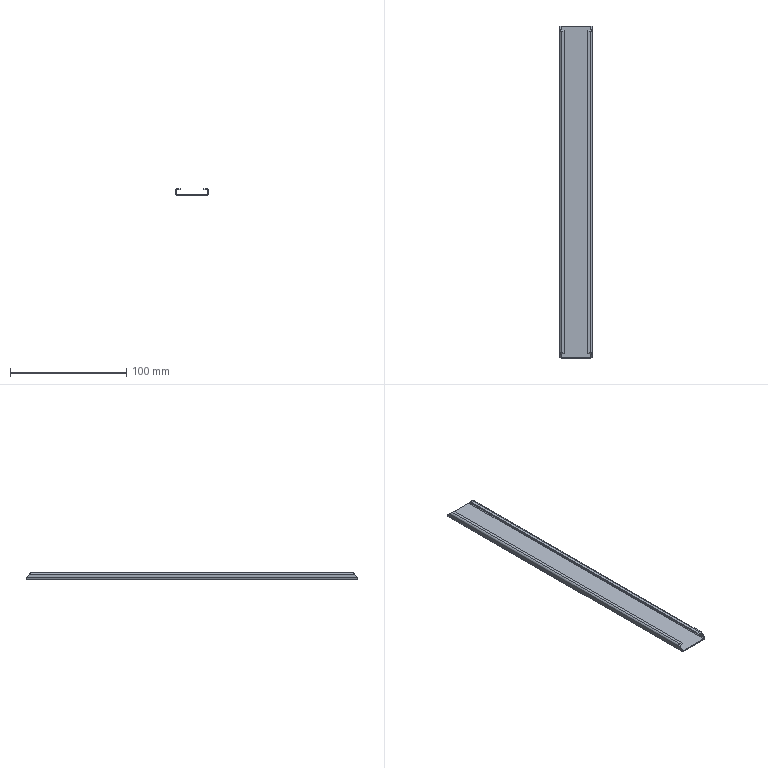Component | SolidWorks | PC-CAJ-P09-1_PM-CAJ-P55-2 | 1 solid | 30 faces | box 28 x 285 x 6 mm | volume 11970 mm3 | plane 22 | cylinder 8 | commonest cylinder face diameters 3 x4 1 x4 | material Plain Carbon Steel
STEP:
#1=COLOUR_RGB('',0.7922,0.8196,0.9333);
#2=FILL_AREA_STYLE_COLOUR('',#1);
#3=FILL_AREA_STYLE('',(#2));
#4=SURFACE_STYLE_FILL_AREA(#3);
#5=SURFACE_SIDE_STYLE('',(#4));
#6=SURFACE_STYLE_USAGE(.BOTH.,#5);
#7=PRESENTATION_STYLE_ASSIGNMENT((#6));
#8=CARTESIAN_POINT('',(6.496,0.5209,3.209));
#9=VERTEX_POINT('',#8);
#10=CARTESIAN_POINT('',(6.496,0.4815,3.169));
#11=VERTEX_POINT('',#10);
#12=CARTESIAN_POINT('',(6.496,0.5209,3.209));
#13=DIRECTION('',(0.,-0.7071,-0.7071));
#14=VECTOR('',#13,39.37);
#15=LINE('',#12,#14);
#16=EDGE_CURVE('',#9,#11,#15,.T.);
#17=ORIENTED_EDGE('',*,*,#16,.F.);
#18=CARTESIAN_POINT('',(6.398,0.5209,3.209));
#19=VERTEX_POINT('',#18);
#20=CARTESIAN_POINT('',(6.417,0.5209,3.209));
#21=DIRECTION('',(-1.,0.,0.));
#22=VECTOR('',#21,39.37);
#23=LINE('',#20,#22);
#24=EDGE_CURVE('',#9,#19,#23,.T.);
#25=ORIENTED_EDGE('',*,*,#24,.T.);
#26=CARTESIAN_POINT('',(6.339,0.4619,3.15));
#27=VERTEX_POINT('',#26);
#28=CARTESIAN_POINT('',(6.398,0.5209,3.209));
#29=CARTESIAN_POINT('',(6.363,0.5209,3.209));
#30=CARTESIAN_POINT('',(6.339,0.4965,3.184));
#31=CARTESIAN_POINT('',(6.339,0.4619,3.15));
#32=(BOUNDED_CURVE()B_SPLINE_CURVE(3,(#28,#29,#30,#31),.UNSPECIFIED.,.F.,.F.)B_SPLINE_CURVE_WITH_KNOTS((4,4),(3.142,4.712),.UNSPECIFIED.)CURVE()GEOMETRIC_REPRESENTATION_ITEM()RATIONAL_B_SPLINE_CURVE((1.,0.8047,0.8047,1.))REPRESENTATION_ITEM(''));
#33=EDGE_CURVE('',#19,#27,#32,.T.);
#34=ORIENTED_EDGE('',*,*,#33,.T.);
#35=CARTESIAN_POINT('',(6.339,0.3438,3.031));
#36=VERTEX_POINT('',#35);
#37=CARTESIAN_POINT('',(6.339,0.4323,3.12));
#38=DIRECTION('',(0.,-0.7071,-0.7071));
#39=VECTOR('',#38,39.37);
#40=LINE('',#37,#39);
#41=EDGE_CURVE('',#27,#36,#40,.T.);
#42=ORIENTED_EDGE('',*,*,#41,.T.);
#43=CARTESIAN_POINT('',(6.378,0.3438,3.031));
#44=VERTEX_POINT('',#43);
#45=CARTESIAN_POINT('',(6.368,0.3438,3.031));
#46=DIRECTION('',(-1.,0.,0.));
#47=VECTOR('',#46,39.37);
#48=LINE('',#45,#47);
#49=EDGE_CURVE('',#44,#36,#48,.T.);
#50=ORIENTED_EDGE('',*,*,#49,.F.);
#51=CARTESIAN_POINT('',(6.378,0.4619,3.15));
#52=VERTEX_POINT('',#51);
#53=CARTESIAN_POINT('',(6.378,0.4323,3.12));
#54=DIRECTION('',(0.,0.7071,0.7071));
#55=VECTOR('',#54,39.37);
#56=LINE('',#53,#55);
#57=EDGE_CURVE('',#44,#52,#56,.T.);
#58=ORIENTED_EDGE('',*,*,#57,.T.);
#59=CARTESIAN_POINT('',(6.398,0.4815,3.169));
#60=VERTEX_POINT('',#59);
#61=CARTESIAN_POINT('',(6.398,0.4815,3.169));
#62=CARTESIAN_POINT('',(6.386,0.4815,3.169));
#63=CARTESIAN_POINT('',(6.378,0.4734,3.161));
#64=CARTESIAN_POINT('',(6.378,0.4619,3.15));
#65=(BOUNDED_CURVE()B_SPLINE_CURVE(3,(#61,#62,#63,#64),.UNSPECIFIED.,.F.,.F.)B_SPLINE_CURVE_WITH_KNOTS((4,4),(0.,1.571),.UNSPECIFIED.)CURVE()GEOMETRIC_REPRESENTATION_ITEM()RATIONAL_B_SPLINE_CURVE((1.,0.8047,0.8047,1.))REPRESENTATION_ITEM(''));
#66=EDGE_CURVE('',#60,#52,#65,.T.);
#67=ORIENTED_EDGE('',*,*,#66,.F.);
#68=CARTESIAN_POINT('',(6.417,0.4815,3.169));
#69=DIRECTION('',(1.,0.,0.));
#70=VECTOR('',#69,39.37);
#71=LINE('',#68,#70);
#72=EDGE_CURVE('',#60,#11,#71,.T.);
#73=ORIENTED_EDGE('',*,*,#72,.T.);
#74=EDGE_LOOP('',(#17,#25,#34,#42,#50,#58,#67,#73));
#75=FACE_OUTER_BOUND('',#74,.T.);
#76=CARTESIAN_POINT('',(6.339,0.5209,3.209));
#77=DIRECTION('',(0.,-0.7071,0.7071));
#78=DIRECTION('',(0.,-0.7071,-0.7071));
#79=AXIS2_PLACEMENT_3D('',#76,#77,#78);
#80=PLANE('',#79);
#81=ADVANCED_FACE('',(#75),#80,.T.);
#82=CARTESIAN_POINT('',(6.496,11.387,3.209));
#83=VERTEX_POINT('',#82);
#84=CARTESIAN_POINT('',(6.398,11.387,3.209));
#85=VERTEX_POINT('',#84);
#86=CARTESIAN_POINT('',(6.447,11.387,3.209));
#87=DIRECTION('',(-1.,0.,-0.));
#88=VECTOR('',#87,39.37);
#89=LINE('',#86,#88);
#90=EDGE_CURVE('',#83,#85,#89,.T.);
#91=ORIENTED_EDGE('',*,*,#90,.T.);
#92=CARTESIAN_POINT('',(6.398,5.954,3.209));
#93=DIRECTION('',(0.,-1.,-0.));
#94=VECTOR('',#93,39.37);
#95=LINE('',#92,#94);
#96=EDGE_CURVE('',#85,#19,#95,.T.);
#97=ORIENTED_EDGE('',*,*,#96,.T.);
#98=ORIENTED_EDGE('',*,*,#24,.F.);
#99=CARTESIAN_POINT('',(6.496,5.954,3.209));
#100=DIRECTION('',(-0.,1.,0.));
#101=VECTOR('',#100,39.37);
#102=LINE('',#99,#101);
#103=EDGE_CURVE('',#9,#83,#102,.T.);
#104=ORIENTED_EDGE('',*,*,#103,.T.);
#105=EDGE_LOOP('',(#91,#97,#98,#104));
#106=FACE_OUTER_BOUND('',#105,.T.);
#107=CARTESIAN_POINT('',(6.398,0.5209,3.209));
#108=DIRECTION('',(0.,-0.,1.));
#109=DIRECTION('',(1.,0.,0.));
#110=AXIS2_PLACEMENT_3D('',#107,#108,#109);
#111=PLANE('',#110);
#112=ADVANCED_FACE('',(#106),#111,.T.);
#113=CARTESIAN_POINT('',(6.398,11.426,3.169));
#114=VERTEX_POINT('',#113);
#115=CARTESIAN_POINT('',(6.496,11.426,3.169));
#116=VERTEX_POINT('',#115);
#117=CARTESIAN_POINT('',(6.447,11.426,3.169));
#118=DIRECTION('',(1.,0.,0.));
#119=VECTOR('',#118,39.37);
#120=LINE('',#117,#119);
#121=EDGE_CURVE('',#114,#116,#120,.T.);
#122=ORIENTED_EDGE('',*,*,#121,.T.);
#123=CARTESIAN_POINT('',(6.496,5.954,3.169));
#124=DIRECTION('',(0.,-1.,-0.));
#125=VECTOR('',#124,39.37);
#126=LINE('',#123,#125);
#127=EDGE_CURVE('',#116,#11,#126,.T.);
#128=ORIENTED_EDGE('',*,*,#127,.T.);
#129=ORIENTED_EDGE('',*,*,#72,.F.);
#130=CARTESIAN_POINT('',(6.398,5.954,3.169));
#131=DIRECTION('',(-0.,1.,0.));
#132=VECTOR('',#131,39.37);
#133=LINE('',#130,#132);
#134=EDGE_CURVE('',#60,#114,#133,.T.);
#135=ORIENTED_EDGE('',*,*,#134,.T.);
#136=EDGE_LOOP('',(#122,#128,#129,#135));
#137=FACE_OUTER_BOUND('',#136,.T.);
#138=CARTESIAN_POINT('',(6.496,0.4815,3.169));
#139=DIRECTION('',(0.,0.,-1.));
#140=DIRECTION('',(-1.,0.,0.));
#141=AXIS2_PLACEMENT_3D('',#138,#139,#140);
#142=PLANE('',#141);
#143=ADVANCED_FACE('',(#137),#142,.T.);
#144=CARTESIAN_POINT('',(6.378,11.564,3.031));
#145=VERTEX_POINT('',#144);
#146=CARTESIAN_POINT('',(6.378,11.446,3.15));
#147=VERTEX_POINT('',#146);
#148=CARTESIAN_POINT('',(6.378,11.564,3.031));
#149=DIRECTION('',(0.,-0.7071,0.7071));
#150=VECTOR('',#149,39.37);
#151=LINE('',#148,#150);
#152=EDGE_CURVE('',#145,#147,#151,.T.);
#153=ORIENTED_EDGE('',*,*,#152,.T.);
#154=CARTESIAN_POINT('',(6.378,5.954,3.15));
#155=DIRECTION('',(0.,-1.,0.));
#156=VECTOR('',#155,39.37);
#157=LINE('',#154,#156);
#158=EDGE_CURVE('',#147,#52,#157,.T.);
#159=ORIENTED_EDGE('',*,*,#158,.T.);
#160=ORIENTED_EDGE('',*,*,#57,.F.);
#161=CARTESIAN_POINT('',(6.378,5.954,3.031));
#162=DIRECTION('',(0.,1.,-0.));
#163=VECTOR('',#162,39.37);
#164=LINE('',#161,#163);
#165=EDGE_CURVE('',#44,#145,#164,.T.);
#166=ORIENTED_EDGE('',*,*,#165,.T.);
#167=EDGE_LOOP('',(#153,#159,#160,#166));
#168=FACE_OUTER_BOUND('',#167,.T.);
#169=CARTESIAN_POINT('',(6.378,0.3438,3.15));
#170=DIRECTION('',(1.,0.,0.));
#171=DIRECTION('',(0.,0.,-1.));
#172=AXIS2_PLACEMENT_3D('',#169,#170,#171);
#173=PLANE('',#172);
#174=ADVANCED_FACE('',(#168),#173,.T.);
#175=CARTESIAN_POINT('',(6.339,11.446,3.15));
#176=VERTEX_POINT('',#175);
#177=CARTESIAN_POINT('',(6.339,11.564,3.031));
#178=VERTEX_POINT('',#177);
#179=CARTESIAN_POINT('',(6.339,11.446,3.15));
#180=DIRECTION('',(0.,0.7071,-0.7071));
#181=VECTOR('',#180,39.37);
#182=LINE('',#179,#181);
#183=EDGE_CURVE('',#176,#178,#182,.T.);
#184=ORIENTED_EDGE('',*,*,#183,.T.);
#185=CARTESIAN_POINT('',(6.339,5.954,3.031));
#186=DIRECTION('',(0.,-1.,0.));
#187=VECTOR('',#186,39.37);
#188=LINE('',#185,#187);
#189=EDGE_CURVE('',#178,#36,#188,.T.);
#190=ORIENTED_EDGE('',*,*,#189,.T.);
#191=ORIENTED_EDGE('',*,*,#41,.F.);
#192=CARTESIAN_POINT('',(6.339,5.954,3.15));
#193=DIRECTION('',(0.,1.,-0.));
#194=VECTOR('',#193,39.37);
#195=LINE('',#192,#194);
#196=EDGE_CURVE('',#27,#176,#195,.T.);
#197=ORIENTED_EDGE('',*,*,#196,.T.);
#198=EDGE_LOOP('',(#184,#190,#191,#197));
#199=FACE_OUTER_BOUND('',#198,.T.);
#200=CARTESIAN_POINT('',(6.339,0.3438,3.031));
#201=DIRECTION('',(-1.,0.,0.));
#202=DIRECTION('',(0.,0.,1.));
#203=AXIS2_PLACEMENT_3D('',#200,#201,#202);
#204=PLANE('',#203);
#205=ADVANCED_FACE('',(#199),#204,.T.);
#206=CARTESIAN_POINT('',(6.398,11.387,3.209));
#207=CARTESIAN_POINT('',(6.363,11.387,3.209));
#208=CARTESIAN_POINT('',(6.339,11.412,3.184));
#209=CARTESIAN_POINT('',(6.339,11.446,3.15));
#210=(BOUNDED_CURVE()B_SPLINE_CURVE(3,(#206,#207,#208,#209),.UNSPECIFIED.,.F.,.F.)B_SPLINE_CURVE_WITH_KNOTS((4,4),(0.,1.571),.UNSPECIFIED.)CURVE()GEOMETRIC_REPRESENTATION_ITEM()RATIONAL_B_SPLINE_CURVE((1.,0.8047,0.8047,1.))REPRESENTATION_ITEM(''));
#211=EDGE_CURVE('',#85,#176,#210,.T.);
#212=ORIENTED_EDGE('',*,*,#211,.T.);
#213=ORIENTED_EDGE('',*,*,#196,.F.);
#214=ORIENTED_EDGE('',*,*,#33,.F.);
#215=ORIENTED_EDGE('',*,*,#96,.F.);
#216=EDGE_LOOP('',(#212,#213,#214,#215));
#217=FACE_OUTER_BOUND('',#216,.T.);
#218=CARTESIAN_POINT('',(6.398,11.446,3.15));
#219=DIRECTION('',(0.,-1.,0.));
#220=DIRECTION('',(0.,0.,-1.));
#221=AXIS2_PLACEMENT_3D('',#218,#219,#220);
#222=CYLINDRICAL_SURFACE('',#221,0.05906);
#223=ADVANCED_FACE('',(#217),#222,.T.);
#224=CARTESIAN_POINT('',(6.368,11.564,3.031));
#225=DIRECTION('',(1.,0.,0.));
#226=VECTOR('',#225,39.37);
#227=LINE('',#224,#226);
#228=EDGE_CURVE('',#178,#145,#227,.T.);
#229=ORIENTED_EDGE('',*,*,#228,.F.);
#230=ORIENTED_EDGE('',*,*,#183,.F.);
#231=ORIENTED_EDGE('',*,*,#211,.F.);
#232=ORIENTED_EDGE('',*,*,#90,.F.);
#233=CARTESIAN_POINT('',(6.496,11.476,3.12));
#234=DIRECTION('',(0.,0.7071,-0.7071));
#235=VECTOR('',#234,39.37);
#236=LINE('',#233,#235);
#237=EDGE_CURVE('',#83,#116,#236,.T.);
#238=ORIENTED_EDGE('',*,*,#237,.T.);
#239=ORIENTED_EDGE('',*,*,#121,.F.);
#240=CARTESIAN_POINT('',(6.398,11.426,3.169));
#241=CARTESIAN_POINT('',(6.386,11.426,3.169));
#242=CARTESIAN_POINT('',(6.378,11.435,3.161));
#243=CARTESIAN_POINT('',(6.378,11.446,3.15));
#244=(BOUNDED_CURVE()B_SPLINE_CURVE(3,(#240,#241,#242,#243),.UNSPECIFIED.,.F.,.F.)B_SPLINE_CURVE_WITH_KNOTS((4,4),(3.142,4.712),.UNSPECIFIED.)CURVE()GEOMETRIC_REPRESENTATION_ITEM()RATIONAL_B_SPLINE_CURVE((1.,0.8047,0.8047,1.))REPRESENTATION_ITEM(''));
#245=EDGE_CURVE('',#114,#147,#244,.T.);
#246=ORIENTED_EDGE('',*,*,#245,.T.);
#247=ORIENTED_EDGE('',*,*,#152,.F.);
#248=EDGE_LOOP('',(#229,#230,#231,#232,#238,#239,#246,#247));
#249=FACE_OUTER_BOUND('',#248,.T.);
#250=CARTESIAN_POINT('',(6.339,11.564,3.031));
#251=DIRECTION('',(0.,0.7071,0.7071));
#252=DIRECTION('',(0.,-0.7071,0.7071));
#253=AXIS2_PLACEMENT_3D('',#250,#251,#252);
#254=PLANE('',#253);
#255=ADVANCED_FACE('',(#249),#254,.T.);
#256=ORIENTED_EDGE('',*,*,#237,.F.);
#257=ORIENTED_EDGE('',*,*,#103,.F.);
#258=ORIENTED_EDGE('',*,*,#16,.T.);
#259=ORIENTED_EDGE('',*,*,#127,.F.);
#260=EDGE_LOOP('',(#256,#257,#258,#259));
#261=FACE_OUTER_BOUND('',#260,.T.);
#262=CARTESIAN_POINT('',(6.496,0.4815,3.209));
#263=DIRECTION('',(1.,0.,0.));
#264=DIRECTION('',(0.,0.,-1.));
#265=AXIS2_PLACEMENT_3D('',#262,#263,#264);
#266=PLANE('',#265);
#267=ADVANCED_FACE('',(#261),#266,.T.);
#268=ORIENTED_EDGE('',*,*,#245,.F.);
#269=ORIENTED_EDGE('',*,*,#134,.F.);
#270=ORIENTED_EDGE('',*,*,#66,.T.);
#271=ORIENTED_EDGE('',*,*,#158,.F.);
#272=EDGE_LOOP('',(#268,#269,#270,#271));
#273=FACE_OUTER_BOUND('',#272,.T.);
#274=CARTESIAN_POINT('',(6.398,0.4619,3.15));
#275=DIRECTION('',(0.,1.,0.));
#276=DIRECTION('',(0.,0.,1.));
#277=AXIS2_PLACEMENT_3D('',#274,#275,#276);
#278=CYLINDRICAL_SURFACE('',#277,0.01969);
#279=ADVANCED_FACE('',(#273),#278,.F.);
#280=CARTESIAN_POINT('',(6.398,0.3438,3.012));
#281=VERTEX_POINT('',#280);
#282=CARTESIAN_POINT('',(6.398,11.564,3.012));
#283=VERTEX_POINT('',#282);
#284=CARTESIAN_POINT('',(6.398,5.954,3.012));
#285=DIRECTION('',(0.,1.,0.));
#286=VECTOR('',#285,39.37);
#287=LINE('',#284,#286);
#288=EDGE_CURVE('',#281,#283,#287,.T.);
#289=ORIENTED_EDGE('',*,*,#288,.T.);
#290=CARTESIAN_POINT('',(6.398,11.564,3.031));
#291=DIRECTION('',(0.,-1.,0.));
#292=DIRECTION('',(0.,0.,1.));
#293=AXIS2_PLACEMENT_3D('',#290,#291,#292);
#294=CIRCLE('',#293,0.01969);
#295=EDGE_CURVE('',#145,#283,#294,.T.);
#296=ORIENTED_EDGE('',*,*,#295,.F.);
#297=ORIENTED_EDGE('',*,*,#165,.F.);
#298=CARTESIAN_POINT('',(6.398,0.3438,3.031));
#299=DIRECTION('',(0.,1.,0.));
#300=DIRECTION('',(0.,0.,1.));
#301=AXIS2_PLACEMENT_3D('',#298,#299,#300);
#302=CIRCLE('',#301,0.01969);
#303=EDGE_CURVE('',#281,#44,#302,.T.);
#304=ORIENTED_EDGE('',*,*,#303,.F.);
#305=EDGE_LOOP('',(#289,#296,#297,#304));
#306=FACE_OUTER_BOUND('',#305,.T.);
#307=CARTESIAN_POINT('',(6.398,0.3438,3.031));
#308=DIRECTION('',(0.,1.,0.));
#309=DIRECTION('',(0.,0.,1.));
#310=AXIS2_PLACEMENT_3D('',#307,#308,#309);
#311=CYLINDRICAL_SURFACE('',#310,0.01969);
#312=ADVANCED_FACE('',(#306),#311,.F.);
#313=CARTESIAN_POINT('',(6.398,11.564,2.972));
#314=VERTEX_POINT('',#313);
#315=CARTESIAN_POINT('',(6.398,0.3438,2.972));
#316=VERTEX_POINT('',#315);
#317=CARTESIAN_POINT('',(6.398,5.954,2.972));
#318=DIRECTION('',(0.,-1.,0.));
#319=VECTOR('',#318,39.37);
#320=LINE('',#317,#319);
#321=EDGE_CURVE('',#314,#316,#320,.T.);
#322=ORIENTED_EDGE('',*,*,#321,.T.);
#323=CARTESIAN_POINT('',(6.398,0.3438,3.031));
#324=DIRECTION('',(0.,1.,0.));
#325=DIRECTION('',(0.,0.,-1.));
#326=AXIS2_PLACEMENT_3D('',#323,#324,#325);
#327=CIRCLE('',#326,0.05906);
#328=EDGE_CURVE('',#316,#36,#327,.T.);
#329=ORIENTED_EDGE('',*,*,#328,.T.);
#330=ORIENTED_EDGE('',*,*,#189,.F.);
#331=CARTESIAN_POINT('',(6.398,11.564,3.031));
#332=DIRECTION('',(0.,-1.,0.));
#333=DIRECTION('',(0.,0.,-1.));
#334=AXIS2_PLACEMENT_3D('',#331,#332,#333);
#335=CIRCLE('',#334,0.05906);
#336=EDGE_CURVE('',#178,#314,#335,.T.);
#337=ORIENTED_EDGE('',*,*,#336,.T.);
#338=EDGE_LOOP('',(#322,#329,#330,#337));
#339=FACE_OUTER_BOUND('',#338,.T.);
#340=CARTESIAN_POINT('',(6.398,11.564,3.031));
#341=DIRECTION('',(0.,-1.,0.));
#342=DIRECTION('',(0.,0.,-1.));
#343=AXIS2_PLACEMENT_3D('',#340,#341,#342);
#344=CYLINDRICAL_SURFACE('',#343,0.05906);
#345=ADVANCED_FACE('',(#339),#344,.T.);
#346=CARTESIAN_POINT('',(7.382,0.3438,3.012));
#347=VERTEX_POINT('',#346);
#348=CARTESIAN_POINT('',(7.382,11.564,3.012));
#349=VERTEX_POINT('',#348);
#350=CARTESIAN_POINT('',(7.382,5.954,3.012));
#351=DIRECTION('',(0.,1.,0.));
#352=VECTOR('',#351,39.37);
#353=LINE('',#350,#352);
#354=EDGE_CURVE('',#347,#349,#353,.T.);
#355=ORIENTED_EDGE('',*,*,#354,.T.);
#356=CARTESIAN_POINT('',(6.89,11.564,3.012));
#357=DIRECTION('',(-1.,0.,0.));
#358=VECTOR('',#357,39.37);
#359=LINE('',#356,#358);
#360=EDGE_CURVE('',#349,#283,#359,.T.);
#361=ORIENTED_EDGE('',*,*,#360,.T.);
#362=ORIENTED_EDGE('',*,*,#288,.F.);
#363=CARTESIAN_POINT('',(6.89,0.3438,3.012));
#364=DIRECTION('',(1.,0.,0.));
#365=VECTOR('',#364,39.37);
#366=LINE('',#363,#365);
#367=EDGE_CURVE('',#281,#347,#366,.T.);
#368=ORIENTED_EDGE('',*,*,#367,.T.);
#369=EDGE_LOOP('',(#355,#361,#362,#368));
#370=FACE_OUTER_BOUND('',#369,.T.);
#371=CARTESIAN_POINT('',(6.398,0.3438,3.012));
#372=DIRECTION('',(0.,0.,1.));
#373=DIRECTION('',(1.,0.,0.));
#374=AXIS2_PLACEMENT_3D('',#371,#372,#373);
#375=PLANE('',#374);
#376=ADVANCED_FACE('',(#370),#375,.T.);
#377=CARTESIAN_POINT('',(6.398,0.3438,3.002));
#378=DIRECTION('',(0.,0.,1.));
#379=VECTOR('',#378,39.37);
#380=LINE('',#377,#379);
#381=EDGE_CURVE('',#316,#281,#380,.T.);
#382=ORIENTED_EDGE('',*,*,#381,.T.);
#383=ORIENTED_EDGE('',*,*,#303,.T.);
#384=ORIENTED_EDGE('',*,*,#49,.T.);
#385=ORIENTED_EDGE('',*,*,#328,.F.);
#386=EDGE_LOOP('',(#382,#383,#384,#385));
#387=FACE_OUTER_BOUND('',#386,.T.);
#388=CARTESIAN_POINT('',(6.339,0.3438,3.031));
#389=DIRECTION('',(0.,-1.,0.));
#390=DIRECTION('',(0.,0.,-1.));
#391=AXIS2_PLACEMENT_3D('',#388,#389,#390);
#392=PLANE('',#391);
#393=ADVANCED_FACE('',(#387),#392,.T.);
#394=CARTESIAN_POINT('',(7.382,11.564,2.972));
#395=VERTEX_POINT('',#394);
#396=CARTESIAN_POINT('',(7.382,0.3438,2.972));
#397=VERTEX_POINT('',#396);
#398=CARTESIAN_POINT('',(7.382,5.954,2.972));
#399=DIRECTION('',(0.,-1.,0.));
#400=VECTOR('',#399,39.37);
#401=LINE('',#398,#400);
#402=EDGE_CURVE('',#395,#397,#401,.T.);
#403=ORIENTED_EDGE('',*,*,#402,.T.);
#404=CARTESIAN_POINT('',(6.89,0.3438,2.972));
#405=DIRECTION('',(-1.,0.,0.));
#406=VECTOR('',#405,39.37);
#407=LINE('',#404,#406);
#408=EDGE_CURVE('',#397,#316,#407,.T.);
#409=ORIENTED_EDGE('',*,*,#408,.T.);
#410=ORIENTED_EDGE('',*,*,#321,.F.);
#411=CARTESIAN_POINT('',(6.89,11.564,2.972));
#412=DIRECTION('',(1.,0.,0.));
#413=VECTOR('',#412,39.37);
#414=LINE('',#411,#413);
#415=EDGE_CURVE('',#314,#395,#414,.T.);
#416=ORIENTED_EDGE('',*,*,#415,.T.);
#417=EDGE_LOOP('',(#403,#409,#410,#416));
#418=FACE_OUTER_BOUND('',#417,.T.);
#419=CARTESIAN_POINT('',(7.382,0.3438,2.972));
#420=DIRECTION('',(0.,0.,-1.));
#421=DIRECTION('',(-1.,0.,0.));
#422=AXIS2_PLACEMENT_3D('',#419,#420,#421);
#423=PLANE('',#422);
#424=ADVANCED_FACE('',(#418),#423,.T.);
#425=CARTESIAN_POINT('',(6.398,11.564,3.002));
#426=DIRECTION('',(0.,0.,-1.));
#427=VECTOR('',#426,39.37);
#428=LINE('',#425,#427);
#429=EDGE_CURVE('',#283,#314,#428,.T.);
#430=ORIENTED_EDGE('',*,*,#429,.T.);
#431=ORIENTED_EDGE('',*,*,#336,.F.);
#432=ORIENTED_EDGE('',*,*,#228,.T.);
#433=ORIENTED_EDGE('',*,*,#295,.T.);
#434=EDGE_LOOP('',(#430,#431,#432,#433));
#435=FACE_OUTER_BOUND('',#434,.T.);
#436=CARTESIAN_POINT('',(6.339,11.564,2.972));
#437=DIRECTION('',(0.,1.,0.));
#438=DIRECTION('',(0.,0.,1.));
#439=AXIS2_PLACEMENT_3D('',#436,#437,#438);
#440=PLANE('',#439);
#441=ADVANCED_FACE('',(#435),#440,.T.);
#442=CARTESIAN_POINT('',(7.382,11.564,3.002));
#443=DIRECTION('',(0.,0.,1.));
#444=VECTOR('',#443,39.37);
#445=LINE('',#442,#444);
#446=EDGE_CURVE('',#395,#349,#445,.T.);
#447=ORIENTED_EDGE('',*,*,#446,.F.);
#448=ORIENTED_EDGE('',*,*,#415,.F.);
#449=ORIENTED_EDGE('',*,*,#429,.F.);
#450=ORIENTED_EDGE('',*,*,#360,.F.);
#451=EDGE_LOOP('',(#447,#448,#449,#450));
#452=FACE_OUTER_BOUND('',#451,.T.);
#453=CARTESIAN_POINT('',(6.398,11.564,2.972));
#454=DIRECTION('',(0.,1.,0.));
#455=DIRECTION('',(0.,0.,1.));
#456=AXIS2_PLACEMENT_3D('',#453,#454,#455);
#457=PLANE('',#456);
#458=ADVANCED_FACE('',(#452),#457,.T.);
#459=ORIENTED_EDGE('',*,*,#354,.F.);
#460=CARTESIAN_POINT('',(7.402,0.3438,3.031));
#461=VERTEX_POINT('',#460);
#462=CARTESIAN_POINT('',(7.382,0.3438,3.031));
#463=DIRECTION('',(0.,1.,0.));
#464=DIRECTION('',(0.,0.,-1.));
#465=AXIS2_PLACEMENT_3D('',#462,#463,#464);
#466=CIRCLE('',#465,0.01969);
#467=EDGE_CURVE('',#461,#347,#466,.T.);
#468=ORIENTED_EDGE('',*,*,#467,.F.);
#469=CARTESIAN_POINT('',(7.402,11.564,3.031));
#470=VERTEX_POINT('',#469);
#471=CARTESIAN_POINT('',(7.402,5.954,3.031));
#472=DIRECTION('',(0.,1.,0.));
#473=VECTOR('',#472,39.37);
#474=LINE('',#471,#473);
#475=EDGE_CURVE('',#461,#470,#474,.T.);
#476=ORIENTED_EDGE('',*,*,#475,.T.);
#477=CARTESIAN_POINT('',(7.382,11.564,3.031));
#478=DIRECTION('',(0.,-1.,0.));
#479=DIRECTION('',(0.,0.,-1.));
#480=AXIS2_PLACEMENT_3D('',#477,#478,#479);
#481=CIRCLE('',#480,0.01969);
#482=EDGE_CURVE('',#349,#470,#481,.T.);
#483=ORIENTED_EDGE('',*,*,#482,.F.);
#484=EDGE_LOOP('',(#459,#468,#476,#483));
#485=FACE_OUTER_BOUND('',#484,.T.);
#486=CARTESIAN_POINT('',(7.382,11.564,3.031));
#487=DIRECTION('',(0.,-1.,0.));
#488=DIRECTION('',(0.,0.,-1.));
#489=AXIS2_PLACEMENT_3D('',#486,#487,#488);
#490=CYLINDRICAL_SURFACE('',#489,0.01969);
#491=ADVANCED_FACE('',(#485),#490,.F.);
#492=CARTESIAN_POINT('',(7.382,0.3438,3.002));
#493=DIRECTION('',(0.,0.,-1.));
#494=VECTOR('',#493,39.37);
#495=LINE('',#492,#494);
#496=EDGE_CURVE('',#347,#397,#495,.T.);
#497=ORIENTED_EDGE('',*,*,#496,.F.);
#498=ORIENTED_EDGE('',*,*,#367,.F.);
#499=ORIENTED_EDGE('',*,*,#381,.F.);
#500=ORIENTED_EDGE('',*,*,#408,.F.);
#501=EDGE_LOOP('',(#497,#498,#499,#500));
#502=FACE_OUTER_BOUND('',#501,.T.);
#503=CARTESIAN_POINT('',(6.398,0.3438,3.012));
#504=DIRECTION('',(0.,-1.,0.));
#505=DIRECTION('',(0.,0.,-1.));
#506=AXIS2_PLACEMENT_3D('',#503,#504,#505);
#507=PLANE('',#506);
#508=ADVANCED_FACE('',(#502),#507,.T.);
#509=ORIENTED_EDGE('',*,*,#402,.F.);
#510=CARTESIAN_POINT('',(7.441,11.564,3.031));
#511=VERTEX_POINT('',#510);
#512=CARTESIAN_POINT('',(7.382,11.564,3.031));
#513=DIRECTION('',(0.,-1.,0.));
#514=DIRECTION('',(0.,0.,1.));
#515=AXIS2_PLACEMENT_3D('',#512,#513,#514);
#516=CIRCLE('',#515,0.05906);
#517=EDGE_CURVE('',#395,#511,#516,.T.);
#518=ORIENTED_EDGE('',*,*,#517,.T.);
#519=CARTESIAN_POINT('',(7.441,0.3438,3.031));
#520=VERTEX_POINT('',#519);
#521=CARTESIAN_POINT('',(7.441,5.954,3.031));
#522=DIRECTION('',(0.,-1.,0.));
#523=VECTOR('',#522,39.37);
#524=LINE('',#521,#523);
#525=EDGE_CURVE('',#511,#520,#524,.T.);
#526=ORIENTED_EDGE('',*,*,#525,.T.);
#527=CARTESIAN_POINT('',(7.382,0.3438,3.031));
#528=DIRECTION('',(0.,1.,0.));
#529=DIRECTION('',(0.,0.,1.));
#530=AXIS2_PLACEMENT_3D('',#527,#528,#529);
#531=CIRCLE('',#530,0.05906);
#532=EDGE_CURVE('',#520,#397,#531,.T.);
#533=ORIENTED_EDGE('',*,*,#532,.T.);
#534=EDGE_LOOP('',(#509,#518,#526,#533));
#535=FACE_OUTER_BOUND('',#534,.T.);
#536=CARTESIAN_POINT('',(7.382,0.3438,3.031));
#537=DIRECTION('',(0.,1.,0.));
#538=DIRECTION('',(0.,0.,1.));
#539=AXIS2_PLACEMENT_3D('',#536,#537,#538);
#540=CYLINDRICAL_SURFACE('',#539,0.05906);
#541=ADVANCED_FACE('',(#535),#540,.T.);
#542=CARTESIAN_POINT('',(7.402,11.446,3.15));
#543=VERTEX_POINT('',#542);
#544=CARTESIAN_POINT('',(7.402,11.446,3.15));
#545=DIRECTION('',(0.,0.7071,-0.7071));
#546=VECTOR('',#545,39.37);
#547=LINE('',#544,#546);
#548=EDGE_CURVE('',#543,#470,#547,.T.);
#549=ORIENTED_EDGE('',*,*,#548,.T.);
#550=ORIENTED_EDGE('',*,*,#475,.F.);
#551=CARTESIAN_POINT('',(7.402,0.4619,3.15));
#552=VERTEX_POINT('',#551);
#553=CARTESIAN_POINT('',(7.402,0.3438,3.031));
#554=DIRECTION('',(0.,0.7071,0.7071));
#555=VECTOR('',#554,39.37);
#556=LINE('',#553,#555);
#557=EDGE_CURVE('',#461,#552,#556,.T.);
#558=ORIENTED_EDGE('',*,*,#557,.T.);
#559=CARTESIAN_POINT('',(7.402,5.954,3.15));
#560=DIRECTION('',(0.,1.,0.));
#561=VECTOR('',#560,39.37);
#562=LINE('',#559,#561);
#563=EDGE_CURVE('',#552,#543,#562,.T.);
#564=ORIENTED_EDGE('',*,*,#563,.T.);
#565=EDGE_LOOP('',(#549,#550,#558,#564));
#566=FACE_OUTER_BOUND('',#565,.T.);
#567=CARTESIAN_POINT('',(7.402,0.3438,3.031));
#568=DIRECTION('',(-1.,0.,0.));
#569=DIRECTION('',(0.,0.,1.));
#570=AXIS2_PLACEMENT_3D('',#567,#568,#569);
#571=PLANE('',#570);
#572=ADVANCED_FACE('',(#566),#571,.T.);
#573=ORIENTED_EDGE('',*,*,#446,.T.);
#574=ORIENTED_EDGE('',*,*,#482,.T.);
#575=CARTESIAN_POINT('',(7.411,11.564,3.031));
#576=DIRECTION('',(1.,0.,0.));
#577=VECTOR('',#576,39.37);
#578=LINE('',#575,#577);
#579=EDGE_CURVE('',#470,#511,#578,.T.);
#580=ORIENTED_EDGE('',*,*,#579,.T.);
#581=ORIENTED_EDGE('',*,*,#517,.F.);
#582=EDGE_LOOP('',(#573,#574,#580,#581));
#583=FACE_OUTER_BOUND('',#582,.T.);
#584=CARTESIAN_POINT('',(7.382,11.564,2.972));
#585=DIRECTION('',(0.,1.,0.));
#586=DIRECTION('',(0.,0.,1.));
#587=AXIS2_PLACEMENT_3D('',#584,#585,#586);
#588=PLANE('',#587);
#589=ADVANCED_FACE('',(#583),#588,.T.);
#590=ORIENTED_EDGE('',*,*,#496,.T.);
#591=ORIENTED_EDGE('',*,*,#532,.F.);
#592=CARTESIAN_POINT('',(7.411,0.3438,3.031));
#593=DIRECTION('',(-1.,0.,0.));
#594=VECTOR('',#593,39.37);
#595=LINE('',#592,#594);
#596=EDGE_CURVE('',#520,#461,#595,.T.);
#597=ORIENTED_EDGE('',*,*,#596,.T.);
#598=ORIENTED_EDGE('',*,*,#467,.T.);
#599=EDGE_LOOP('',(#590,#591,#597,#598));
#600=FACE_OUTER_BOUND('',#599,.T.);
#601=CARTESIAN_POINT('',(7.382,0.3438,3.031));
#602=DIRECTION('',(0.,-1.,0.));
#603=DIRECTION('',(0.,0.,-1.));
#604=AXIS2_PLACEMENT_3D('',#601,#602,#603);
#605=PLANE('',#604);
#606=ADVANCED_FACE('',(#600),#605,.T.);
#607=CARTESIAN_POINT('',(7.441,11.446,3.15));
#608=VERTEX_POINT('',#607);
#609=CARTESIAN_POINT('',(7.441,11.564,3.031));
#610=DIRECTION('',(0.,-0.7071,0.7071));
#611=VECTOR('',#610,39.37);
#612=LINE('',#609,#611);
#613=EDGE_CURVE('',#511,#608,#612,.T.);
#614=ORIENTED_EDGE('',*,*,#613,.T.);
#615=CARTESIAN_POINT('',(7.441,0.4619,3.15));
#616=VERTEX_POINT('',#615);
#617=CARTESIAN_POINT('',(7.441,5.954,3.15));
#618=DIRECTION('',(0.,-1.,-0.));
#619=VECTOR('',#618,39.37);
#620=LINE('',#617,#619);
#621=EDGE_CURVE('',#608,#616,#620,.T.);
#622=ORIENTED_EDGE('',*,*,#621,.T.);
#623=CARTESIAN_POINT('',(7.441,0.4619,3.15));
#624=DIRECTION('',(0.,-0.7071,-0.7071));
#625=VECTOR('',#624,39.37);
#626=LINE('',#623,#625);
#627=EDGE_CURVE('',#616,#520,#626,.T.);
#628=ORIENTED_EDGE('',*,*,#627,.T.);
#629=ORIENTED_EDGE('',*,*,#525,.F.);
#630=EDGE_LOOP('',(#614,#622,#628,#629));
#631=FACE_OUTER_BOUND('',#630,.T.);
#632=CARTESIAN_POINT('',(7.441,0.3438,3.15));
#633=DIRECTION('',(1.,0.,0.));
#634=DIRECTION('',(0.,0.,-1.));
#635=AXIS2_PLACEMENT_3D('',#632,#633,#634);
#636=PLANE('',#635);
#637=ADVANCED_FACE('',(#631),#636,.T.);
#638=CARTESIAN_POINT('',(7.283,11.387,3.209));
#639=VERTEX_POINT('',#638);
#640=CARTESIAN_POINT('',(7.382,11.387,3.209));
#641=VERTEX_POINT('',#640);
#642=CARTESIAN_POINT('',(7.362,11.387,3.209));
#643=DIRECTION('',(1.,0.,-0.));
#644=VECTOR('',#643,39.37);
#645=LINE('',#642,#644);
#646=EDGE_CURVE('',#639,#641,#645,.T.);
#647=ORIENTED_EDGE('',*,*,#646,.T.);
#648=CARTESIAN_POINT('',(7.382,11.387,3.209));
#649=CARTESIAN_POINT('',(7.416,11.387,3.209));
#650=CARTESIAN_POINT('',(7.441,11.412,3.184));
#651=CARTESIAN_POINT('',(7.441,11.446,3.15));
#652=(BOUNDED_CURVE()B_SPLINE_CURVE(3,(#648,#649,#650,#651),.UNSPECIFIED.,.F.,.T.)B_SPLINE_CURVE_WITH_KNOTS((4,4),(3.142,4.712),.UNSPECIFIED.)CURVE()GEOMETRIC_REPRESENTATION_ITEM()RATIONAL_B_SPLINE_CURVE((1.,0.8047,0.8047,1.))REPRESENTATION_ITEM(''));
#653=EDGE_CURVE('',#641,#608,#652,.T.);
#654=ORIENTED_EDGE('',*,*,#653,.T.);
#655=ORIENTED_EDGE('',*,*,#613,.F.);
#656=ORIENTED_EDGE('',*,*,#579,.F.);
#657=ORIENTED_EDGE('',*,*,#548,.F.);
#658=CARTESIAN_POINT('',(7.382,11.426,3.169));
#659=VERTEX_POINT('',#658);
#660=CARTESIAN_POINT('',(7.402,11.446,3.15));
#661=CARTESIAN_POINT('',(7.402,11.435,3.161));
#662=CARTESIAN_POINT('',(7.393,11.426,3.169));
#663=CARTESIAN_POINT('',(7.382,11.426,3.169));
#664=(BOUNDED_CURVE()B_SPLINE_CURVE(3,(#660,#661,#662,#663),.UNSPECIFIED.,.F.,.F.)B_SPLINE_CURVE_WITH_KNOTS((4,4),(4.712,6.283),.UNSPECIFIED.)CURVE()GEOMETRIC_REPRESENTATION_ITEM()RATIONAL_B_SPLINE_CURVE((1.,0.8047,0.8047,1.))REPRESENTATION_ITEM(''));
#665=EDGE_CURVE('',#543,#659,#664,.T.);
#666=ORIENTED_EDGE('',*,*,#665,.T.);
#667=CARTESIAN_POINT('',(7.283,11.426,3.169));
#668=VERTEX_POINT('',#667);
#669=CARTESIAN_POINT('',(7.362,11.426,3.169));
#670=DIRECTION('',(-1.,0.,0.));
#671=VECTOR('',#670,39.37);
#672=LINE('',#669,#671);
#673=EDGE_CURVE('',#659,#668,#672,.T.);
#674=ORIENTED_EDGE('',*,*,#673,.T.);
#675=CARTESIAN_POINT('',(7.283,11.387,3.209));
#676=DIRECTION('',(-0.,0.7071,-0.7071));
#677=VECTOR('',#676,39.37);
#678=LINE('',#675,#677);
#679=EDGE_CURVE('',#639,#668,#678,.T.);
#680=ORIENTED_EDGE('',*,*,#679,.F.);
#681=EDGE_LOOP('',(#647,#654,#655,#656,#657,#666,#674,#680));
#682=FACE_OUTER_BOUND('',#681,.T.);
#683=CARTESIAN_POINT('',(7.283,11.564,3.031));
#684=DIRECTION('',(0.,0.7071,0.7071));
#685=DIRECTION('',(0.,-0.7071,0.7071));
#686=AXIS2_PLACEMENT_3D('',#683,#684,#685);
#687=PLANE('',#686);
#688=ADVANCED_FACE('',(#682),#687,.T.);
#689=ORIENTED_EDGE('',*,*,#665,.F.);
#690=ORIENTED_EDGE('',*,*,#563,.F.);
#691=CARTESIAN_POINT('',(7.382,0.4815,3.169));
#692=VERTEX_POINT('',#691);
#693=CARTESIAN_POINT('',(7.402,0.4619,3.15));
#694=CARTESIAN_POINT('',(7.402,0.4734,3.161));
#695=CARTESIAN_POINT('',(7.393,0.4815,3.169));
#696=CARTESIAN_POINT('',(7.382,0.4815,3.169));
#697=(BOUNDED_CURVE()B_SPLINE_CURVE(3,(#693,#694,#695,#696),.UNSPECIFIED.,.F.,.F.)B_SPLINE_CURVE_WITH_KNOTS((4,4),(1.571,3.142),.UNSPECIFIED.)CURVE()GEOMETRIC_REPRESENTATION_ITEM()RATIONAL_B_SPLINE_CURVE((1.,0.8047,0.8047,1.))REPRESENTATION_ITEM(''));
#698=EDGE_CURVE('',#552,#692,#697,.T.);
#699=ORIENTED_EDGE('',*,*,#698,.T.);
#700=CARTESIAN_POINT('',(7.382,5.954,3.169));
#701=DIRECTION('',(0.,1.,-0.));
#702=VECTOR('',#701,39.37);
#703=LINE('',#700,#702);
#704=EDGE_CURVE('',#692,#659,#703,.T.);
#705=ORIENTED_EDGE('',*,*,#704,.T.);
#706=EDGE_LOOP('',(#689,#690,#699,#705));
#707=FACE_OUTER_BOUND('',#706,.T.);
#708=CARTESIAN_POINT('',(7.382,11.446,3.15));
#709=DIRECTION('',(0.,-1.,0.));
#710=DIRECTION('',(0.,0.,-1.));
#711=AXIS2_PLACEMENT_3D('',#708,#709,#710);
#712=CYLINDRICAL_SURFACE('',#711,0.01969);
#713=ADVANCED_FACE('',(#707),#712,.F.);
#714=ORIENTED_EDGE('',*,*,#557,.F.);
#715=ORIENTED_EDGE('',*,*,#596,.F.);
#716=ORIENTED_EDGE('',*,*,#627,.F.);
#717=CARTESIAN_POINT('',(7.382,0.5209,3.209));
#718=VERTEX_POINT('',#717);
#719=CARTESIAN_POINT('',(7.441,0.4619,3.15));
#720=CARTESIAN_POINT('',(7.441,0.4965,3.184));
#721=CARTESIAN_POINT('',(7.416,0.5209,3.209));
#722=CARTESIAN_POINT('',(7.382,0.5209,3.209));
#723=(BOUNDED_CURVE()B_SPLINE_CURVE(3,(#719,#720,#721,#722),.UNSPECIFIED.,.F.,.F.)B_SPLINE_CURVE_WITH_KNOTS((4,4),(4.712,6.283),.UNSPECIFIED.)CURVE()GEOMETRIC_REPRESENTATION_ITEM()RATIONAL_B_SPLINE_CURVE((1.,0.8047,0.8047,1.))REPRESENTATION_ITEM(''));
#724=EDGE_CURVE('',#616,#718,#723,.T.);
#725=ORIENTED_EDGE('',*,*,#724,.T.);
#726=CARTESIAN_POINT('',(7.283,0.5209,3.209));
#727=VERTEX_POINT('',#726);
#728=CARTESIAN_POINT('',(7.362,0.5209,3.209));
#729=DIRECTION('',(-1.,0.,0.));
#730=VECTOR('',#729,39.37);
#731=LINE('',#728,#730);
#732=EDGE_CURVE('',#718,#727,#731,.T.);
#733=ORIENTED_EDGE('',*,*,#732,.T.);
#734=CARTESIAN_POINT('',(7.283,0.4815,3.169));
#735=VERTEX_POINT('',#734);
#736=CARTESIAN_POINT('',(7.283,0.4815,3.169));
#737=DIRECTION('',(0.,0.7071,0.7071));
#738=VECTOR('',#737,39.37);
#739=LINE('',#736,#738);
#740=EDGE_CURVE('',#735,#727,#739,.T.);
#741=ORIENTED_EDGE('',*,*,#740,.F.);
#742=CARTESIAN_POINT('',(7.362,0.4815,3.169));
#743=DIRECTION('',(1.,0.,-0.));
#744=VECTOR('',#743,39.37);
#745=LINE('',#742,#744);
#746=EDGE_CURVE('',#735,#692,#745,.T.);
#747=ORIENTED_EDGE('',*,*,#746,.T.);
#748=ORIENTED_EDGE('',*,*,#698,.F.);
#749=EDGE_LOOP('',(#714,#715,#716,#725,#733,#741,#747,#748));
#750=FACE_OUTER_BOUND('',#749,.T.);
#751=CARTESIAN_POINT('',(7.283,0.5209,3.209));
#752=DIRECTION('',(0.,-0.7071,0.7071));
#753=DIRECTION('',(-0.,-0.7071,-0.7071));
#754=AXIS2_PLACEMENT_3D('',#751,#752,#753);
#755=PLANE('',#754);
#756=ADVANCED_FACE('',(#750),#755,.T.);
#757=ORIENTED_EDGE('',*,*,#653,.F.);
#758=CARTESIAN_POINT('',(7.382,5.954,3.209));
#759=DIRECTION('',(0.,-1.,0.));
#760=VECTOR('',#759,39.37);
#761=LINE('',#758,#760);
#762=EDGE_CURVE('',#641,#718,#761,.T.);
#763=ORIENTED_EDGE('',*,*,#762,.T.);
#764=ORIENTED_EDGE('',*,*,#724,.F.);
#765=ORIENTED_EDGE('',*,*,#621,.F.);
#766=EDGE_LOOP('',(#757,#763,#764,#765));
#767=FACE_OUTER_BOUND('',#766,.T.);
#768=CARTESIAN_POINT('',(7.382,0.4619,3.15));
#769=DIRECTION('',(0.,1.,0.));
#770=DIRECTION('',(0.,0.,1.));
#771=AXIS2_PLACEMENT_3D('',#768,#769,#770);
#772=CYLINDRICAL_SURFACE('',#771,0.05906);
#773=ADVANCED_FACE('',(#767),#772,.T.);
#774=ORIENTED_EDGE('',*,*,#646,.F.);
#775=CARTESIAN_POINT('',(7.283,5.954,3.209));
#776=DIRECTION('',(0.,-1.,0.));
#777=VECTOR('',#776,39.37);
#778=LINE('',#775,#777);
#779=EDGE_CURVE('',#639,#727,#778,.T.);
#780=ORIENTED_EDGE('',*,*,#779,.T.);
#781=ORIENTED_EDGE('',*,*,#732,.F.);
#782=ORIENTED_EDGE('',*,*,#762,.F.);
#783=EDGE_LOOP('',(#774,#780,#781,#782));
#784=FACE_OUTER_BOUND('',#783,.T.);
#785=CARTESIAN_POINT('',(7.283,0.5209,3.209));
#786=DIRECTION('',(0.,0.,1.));
#787=DIRECTION('',(1.,0.,-0.));
#788=AXIS2_PLACEMENT_3D('',#785,#786,#787);
#789=PLANE('',#788);
#790=ADVANCED_FACE('',(#784),#789,.T.);
#791=ORIENTED_EDGE('',*,*,#673,.F.);
#792=ORIENTED_EDGE('',*,*,#704,.F.);
#793=ORIENTED_EDGE('',*,*,#746,.F.);
#794=CARTESIAN_POINT('',(7.283,5.954,3.169));
#795=DIRECTION('',(-0.,1.,-0.));
#796=VECTOR('',#795,39.37);
#797=LINE('',#794,#796);
#798=EDGE_CURVE('',#735,#668,#797,.T.);
#799=ORIENTED_EDGE('',*,*,#798,.T.);
#800=EDGE_LOOP('',(#791,#792,#793,#799));
#801=FACE_OUTER_BOUND('',#800,.T.);
#802=CARTESIAN_POINT('',(7.382,0.4815,3.169));
#803=DIRECTION('',(-0.,-0.,-1.));
#804=DIRECTION('',(-1.,0.,0.));
#805=AXIS2_PLACEMENT_3D('',#802,#803,#804);
#806=PLANE('',#805);
#807=ADVANCED_FACE('',(#801),#806,.T.);
#808=ORIENTED_EDGE('',*,*,#679,.T.);
#809=ORIENTED_EDGE('',*,*,#798,.F.);
#810=ORIENTED_EDGE('',*,*,#740,.T.);
#811=ORIENTED_EDGE('',*,*,#779,.F.);
#812=EDGE_LOOP('',(#808,#809,#810,#811));
#813=FACE_OUTER_BOUND('',#812,.T.);
#814=CARTESIAN_POINT('',(7.283,0.4815,3.169));
#815=DIRECTION('',(-1.,-0.,0.));
#816=DIRECTION('',(0.,0.,1.));
#817=AXIS2_PLACEMENT_3D('',#814,#815,#816);
#818=PLANE('',#817);
#819=ADVANCED_FACE('',(#813),#818,.T.);
#820=CLOSED_SHELL('',(#81,#112,#143,#174,#205,#223,#255,#267,#279,#312,#345,#376,#393,#424,#441,#458,#491,#508,#541,#572,#589,#606,#637,#688,#713,#756,#773,#790,#807,#819));
#821=MANIFOLD_SOLID_BREP('',#820);
#822=STYLED_ITEM('',(#7),#821);
#823=PRESENTATION_LAYER_ASSIGNMENT('','',(#822));
#824=(LENGTH_UNIT()NAMED_UNIT(*)SI_UNIT($,.METRE.));
#825=LENGTH_MEASURE_WITH_UNIT(LENGTH_MEASURE(0.0254),#824);
#826=DIMENSIONAL_EXPONENTS(1.,0.,0.,0.,0.,0.,0.);
#827=(CONVERSION_BASED_UNIT('',#825)LENGTH_UNIT()NAMED_UNIT(#826));
#828=UNCERTAINTY_MEASURE_WITH_UNIT(LENGTH_MEASURE(0.00001),#827,'','');
#829=(NAMED_UNIT(*)PLANE_ANGLE_UNIT()SI_UNIT($,.RADIAN.));
#830=(NAMED_UNIT(*)SI_UNIT($,.STERADIAN.)SOLID_ANGLE_UNIT());
#831=(GEOMETRIC_REPRESENTATION_CONTEXT(3)GLOBAL_UNCERTAINTY_ASSIGNED_CONTEXT((#828))GLOBAL_UNIT_ASSIGNED_CONTEXT((#827,#829,#830))REPRESENTATION_CONTEXT('',''));
#832=MECHANICAL_DESIGN_GEOMETRIC_PRESENTATION_REPRESENTATION('',(#822),#831);
#833=CARTESIAN_POINT('',(0.,0.,0.));
#834=DIRECTION('',(0.,0.,1.));
#835=DIRECTION('',(1.,0.,0.));
#836=AXIS2_PLACEMENT_3D('',#833,#834,#835);
#837=(LENGTH_UNIT()NAMED_UNIT(*)SI_UNIT($,.METRE.));
#838=LENGTH_MEASURE_WITH_UNIT(LENGTH_MEASURE(0.0254),#837);
#839=DIMENSIONAL_EXPONENTS(1.,0.,0.,0.,0.,0.,0.);
#840=(CONVERSION_BASED_UNIT('',#838)LENGTH_UNIT()NAMED_UNIT(#839));
#841=UNCERTAINTY_MEASURE_WITH_UNIT(LENGTH_MEASURE(0.00001),#840,'','');
#842=(NAMED_UNIT(*)PLANE_ANGLE_UNIT()SI_UNIT($,.RADIAN.));
#843=(NAMED_UNIT(*)SI_UNIT($,.STERADIAN.)SOLID_ANGLE_UNIT());
#844=(GEOMETRIC_REPRESENTATION_CONTEXT(3)GLOBAL_UNCERTAINTY_ASSIGNED_CONTEXT((#841))GLOBAL_UNIT_ASSIGNED_CONTEXT((#840,#842,#843))REPRESENTATION_CONTEXT('',''));
#845=ADVANCED_BREP_SHAPE_REPRESENTATION('',(#821,#836),#844);